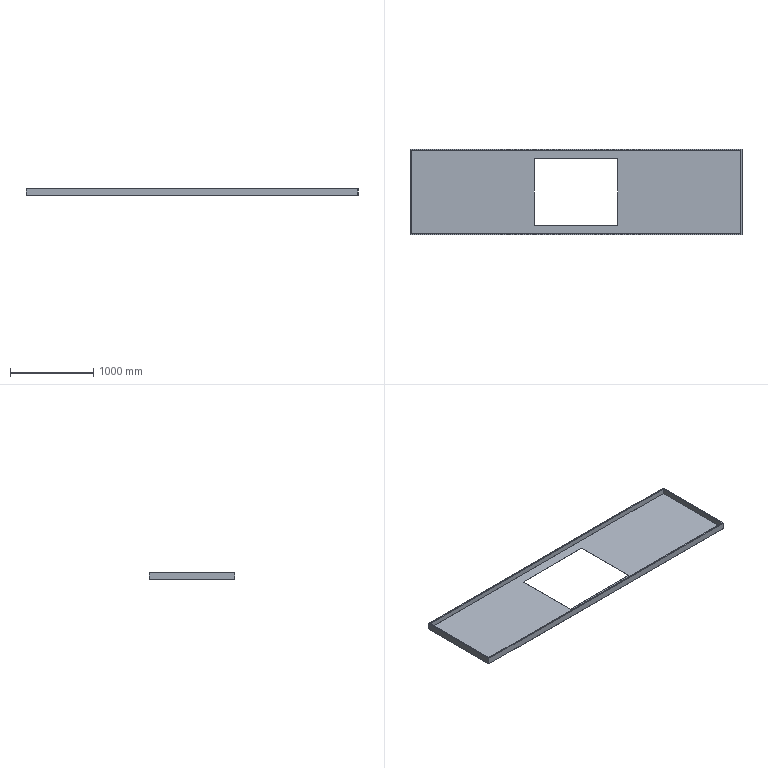Component | NX | DB7_2 | 1 solid | 20 faces | volume 6348027 mm3 | plane 20